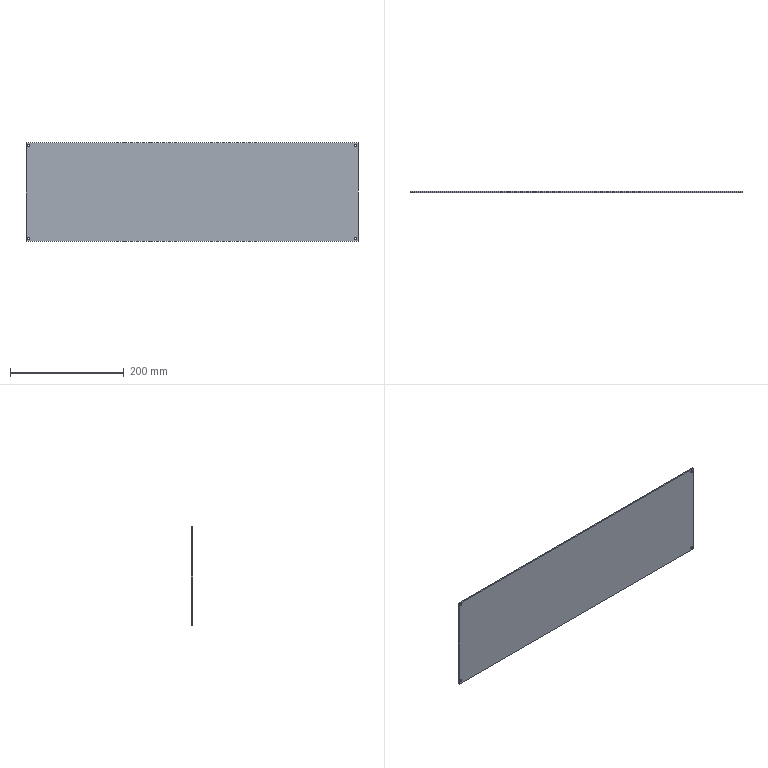Component | SolidWorks | TransformerBoxAssembly-1_ElectricalBoxTopPlate-1 | 1 solid | 14 faces | box 583 x 2 x 173 mm | volume 201617 mm3 | cylinder 8 | plane 6 | commonest cylinder face diameters 4 x8
build123d program:
from build123d import *

# Parameters (mm, degrees)
SKETCH1_W           = 583
SKETCH1_H           = 173
SKETCH1_R           = 2
BOSS_EXTRUDE1_DEPTH = 2


with BuildPart() as part:
    # Sketch1 → Boss-Extrude1 (new body)
    with BuildSketch(Plane.XY):
        with Locations((239.686, -61.336)):
            Rectangle(SKETCH1_W, SKETCH1_H)
        with Locations((-46.814, 20.164)):
            Circle(SKETCH1_R, mode=Mode.SUBTRACT)
        with Locations((-46.814, -142.836)):
            Circle(SKETCH1_R, mode=Mode.SUBTRACT)
        with Locations((526.186, 20.164)):
            Circle(SKETCH1_R, mode=Mode.SUBTRACT)
        with Locations((526.186, -142.836)):
            Circle(SKETCH1_R, mode=Mode.SUBTRACT)
    extrude(amount=BOSS_EXTRUDE1_DEPTH)


solid = part.part

# Placed as in the assembly
solid = solid.moved(Location((-831.736, 541.566, -524.683), (90, 0, 0)))
STEP:
#1=COLOUR_RGB('',0.7922,0.8196,0.9333);
#2=FILL_AREA_STYLE_COLOUR('',#1);
#3=FILL_AREA_STYLE('',(#2));
#4=SURFACE_STYLE_FILL_AREA(#3);
#5=SURFACE_SIDE_STYLE('',(#4));
#6=SURFACE_STYLE_USAGE(.BOTH.,#5);
#7=PRESENTATION_STYLE_ASSIGNMENT((#6));
#8=CARTESIAN_POINT('',(-34.51,21.243,-19.863));
#9=VERTEX_POINT('',#8);
#10=CARTESIAN_POINT('',(-34.667,21.243,-19.863));
#11=VERTEX_POINT('',#10);
#12=CARTESIAN_POINT('',(-34.589,21.243,-19.863));
#13=DIRECTION('',(-0.,-1.,-0.));
#14=DIRECTION('',(-1.,0.,0.));
#15=AXIS2_PLACEMENT_3D('',#12,#13,#14);
#16=CIRCLE('',#15,0.07874);
#17=EDGE_CURVE('',#9,#11,#16,.T.);
#18=ORIENTED_EDGE('',*,*,#17,.T.);
#19=CARTESIAN_POINT('',(-34.667,21.322,-19.863));
#20=VERTEX_POINT('',#19);
#21=CARTESIAN_POINT('',(-34.667,21.243,-19.863));
#22=DIRECTION('',(0.,1.,0.));
#23=VECTOR('',#22,39.37);
#24=LINE('',#21,#23);
#25=EDGE_CURVE('',#11,#20,#24,.T.);
#26=ORIENTED_EDGE('',*,*,#25,.T.);
#27=CARTESIAN_POINT('',(-34.51,21.322,-19.863));
#28=VERTEX_POINT('',#27);
#29=CARTESIAN_POINT('',(-34.589,21.322,-19.863));
#30=DIRECTION('',(-0.,-1.,-0.));
#31=DIRECTION('',(-1.,0.,0.));
#32=AXIS2_PLACEMENT_3D('',#29,#30,#31);
#33=CIRCLE('',#32,0.07874);
#34=EDGE_CURVE('',#28,#20,#33,.T.);
#35=ORIENTED_EDGE('',*,*,#34,.F.);
#36=CARTESIAN_POINT('',(-34.51,21.243,-19.863));
#37=DIRECTION('',(0.,1.,0.));
#38=VECTOR('',#37,39.37);
#39=LINE('',#36,#38);
#40=EDGE_CURVE('',#9,#28,#39,.T.);
#41=ORIENTED_EDGE('',*,*,#40,.F.);
#42=EDGE_LOOP('',(#18,#26,#35,#41));
#43=FACE_OUTER_BOUND('',#42,.T.);
#44=CARTESIAN_POINT('',(-34.589,21.243,-19.863));
#45=DIRECTION('',(0.,1.,0.));
#46=DIRECTION('',(1.,0.,0.));
#47=AXIS2_PLACEMENT_3D('',#44,#45,#46);
#48=CYLINDRICAL_SURFACE('',#47,0.07874);
#49=ADVANCED_FACE('',(#43),#48,.F.);
#50=CARTESIAN_POINT('',(-34.51,21.243,-26.28));
#51=VERTEX_POINT('',#50);
#52=CARTESIAN_POINT('',(-34.667,21.243,-26.28));
#53=VERTEX_POINT('',#52);
#54=CARTESIAN_POINT('',(-34.589,21.243,-26.28));
#55=DIRECTION('',(-0.,-1.,-0.));
#56=DIRECTION('',(-1.,0.,0.));
#57=AXIS2_PLACEMENT_3D('',#54,#55,#56);
#58=CIRCLE('',#57,0.07874);
#59=EDGE_CURVE('',#51,#53,#58,.T.);
#60=ORIENTED_EDGE('',*,*,#59,.T.);
#61=CARTESIAN_POINT('',(-34.667,21.322,-26.28));
#62=VERTEX_POINT('',#61);
#63=CARTESIAN_POINT('',(-34.667,21.243,-26.28));
#64=DIRECTION('',(0.,1.,0.));
#65=VECTOR('',#64,39.37);
#66=LINE('',#63,#65);
#67=EDGE_CURVE('',#53,#62,#66,.T.);
#68=ORIENTED_EDGE('',*,*,#67,.T.);
#69=CARTESIAN_POINT('',(-34.51,21.322,-26.28));
#70=VERTEX_POINT('',#69);
#71=CARTESIAN_POINT('',(-34.589,21.322,-26.28));
#72=DIRECTION('',(-0.,-1.,-0.));
#73=DIRECTION('',(-1.,0.,0.));
#74=AXIS2_PLACEMENT_3D('',#71,#72,#73);
#75=CIRCLE('',#74,0.07874);
#76=EDGE_CURVE('',#70,#62,#75,.T.);
#77=ORIENTED_EDGE('',*,*,#76,.F.);
#78=CARTESIAN_POINT('',(-34.51,21.243,-26.28));
#79=DIRECTION('',(0.,1.,0.));
#80=VECTOR('',#79,39.37);
#81=LINE('',#78,#80);
#82=EDGE_CURVE('',#51,#70,#81,.T.);
#83=ORIENTED_EDGE('',*,*,#82,.F.);
#84=EDGE_LOOP('',(#60,#68,#77,#83));
#85=FACE_OUTER_BOUND('',#84,.T.);
#86=CARTESIAN_POINT('',(-34.589,21.243,-26.28));
#87=DIRECTION('',(0.,1.,0.));
#88=DIRECTION('',(1.,0.,0.));
#89=AXIS2_PLACEMENT_3D('',#86,#87,#88);
#90=CYLINDRICAL_SURFACE('',#89,0.07874);
#91=ADVANCED_FACE('',(#85),#90,.F.);
#92=CARTESIAN_POINT('',(-11.951,21.243,-19.863));
#93=VERTEX_POINT('',#92);
#94=CARTESIAN_POINT('',(-12.108,21.243,-19.863));
#95=VERTEX_POINT('',#94);
#96=CARTESIAN_POINT('',(-12.03,21.243,-19.863));
#97=DIRECTION('',(-0.,-1.,-0.));
#98=DIRECTION('',(-1.,0.,0.));
#99=AXIS2_PLACEMENT_3D('',#96,#97,#98);
#100=CIRCLE('',#99,0.07874);
#101=EDGE_CURVE('',#93,#95,#100,.T.);
#102=ORIENTED_EDGE('',*,*,#101,.T.);
#103=CARTESIAN_POINT('',(-12.108,21.322,-19.863));
#104=VERTEX_POINT('',#103);
#105=CARTESIAN_POINT('',(-12.108,21.243,-19.863));
#106=DIRECTION('',(0.,1.,0.));
#107=VECTOR('',#106,39.37);
#108=LINE('',#105,#107);
#109=EDGE_CURVE('',#95,#104,#108,.T.);
#110=ORIENTED_EDGE('',*,*,#109,.T.);
#111=CARTESIAN_POINT('',(-11.951,21.322,-19.863));
#112=VERTEX_POINT('',#111);
#113=CARTESIAN_POINT('',(-12.03,21.322,-19.863));
#114=DIRECTION('',(-0.,-1.,-0.));
#115=DIRECTION('',(-1.,0.,0.));
#116=AXIS2_PLACEMENT_3D('',#113,#114,#115);
#117=CIRCLE('',#116,0.07874);
#118=EDGE_CURVE('',#112,#104,#117,.T.);
#119=ORIENTED_EDGE('',*,*,#118,.F.);
#120=CARTESIAN_POINT('',(-11.951,21.243,-19.863));
#121=DIRECTION('',(0.,1.,0.));
#122=VECTOR('',#121,39.37);
#123=LINE('',#120,#122);
#124=EDGE_CURVE('',#93,#112,#123,.T.);
#125=ORIENTED_EDGE('',*,*,#124,.F.);
#126=EDGE_LOOP('',(#102,#110,#119,#125));
#127=FACE_OUTER_BOUND('',#126,.T.);
#128=CARTESIAN_POINT('',(-12.03,21.243,-19.863));
#129=DIRECTION('',(0.,1.,0.));
#130=DIRECTION('',(1.,0.,0.));
#131=AXIS2_PLACEMENT_3D('',#128,#129,#130);
#132=CYLINDRICAL_SURFACE('',#131,0.07874);
#133=ADVANCED_FACE('',(#127),#132,.F.);
#134=CARTESIAN_POINT('',(-11.951,21.243,-26.28));
#135=VERTEX_POINT('',#134);
#136=CARTESIAN_POINT('',(-12.108,21.243,-26.28));
#137=VERTEX_POINT('',#136);
#138=CARTESIAN_POINT('',(-12.03,21.243,-26.28));
#139=DIRECTION('',(-0.,-1.,-0.));
#140=DIRECTION('',(-1.,0.,0.));
#141=AXIS2_PLACEMENT_3D('',#138,#139,#140);
#142=CIRCLE('',#141,0.07874);
#143=EDGE_CURVE('',#135,#137,#142,.T.);
#144=ORIENTED_EDGE('',*,*,#143,.T.);
#145=CARTESIAN_POINT('',(-12.108,21.322,-26.28));
#146=VERTEX_POINT('',#145);
#147=CARTESIAN_POINT('',(-12.108,21.243,-26.28));
#148=DIRECTION('',(0.,1.,0.));
#149=VECTOR('',#148,39.37);
#150=LINE('',#147,#149);
#151=EDGE_CURVE('',#137,#146,#150,.T.);
#152=ORIENTED_EDGE('',*,*,#151,.T.);
#153=CARTESIAN_POINT('',(-11.951,21.322,-26.28));
#154=VERTEX_POINT('',#153);
#155=CARTESIAN_POINT('',(-12.03,21.322,-26.28));
#156=DIRECTION('',(-0.,-1.,-0.));
#157=DIRECTION('',(-1.,0.,0.));
#158=AXIS2_PLACEMENT_3D('',#155,#156,#157);
#159=CIRCLE('',#158,0.07874);
#160=EDGE_CURVE('',#154,#146,#159,.T.);
#161=ORIENTED_EDGE('',*,*,#160,.F.);
#162=CARTESIAN_POINT('',(-11.951,21.243,-26.28));
#163=DIRECTION('',(0.,1.,0.));
#164=VECTOR('',#163,39.37);
#165=LINE('',#162,#164);
#166=EDGE_CURVE('',#135,#154,#165,.T.);
#167=ORIENTED_EDGE('',*,*,#166,.F.);
#168=EDGE_LOOP('',(#144,#152,#161,#167));
#169=FACE_OUTER_BOUND('',#168,.T.);
#170=CARTESIAN_POINT('',(-12.03,21.243,-26.28));
#171=DIRECTION('',(0.,1.,0.));
#172=DIRECTION('',(1.,0.,0.));
#173=AXIS2_PLACEMENT_3D('',#170,#171,#172);
#174=CYLINDRICAL_SURFACE('',#173,0.07874);
#175=ADVANCED_FACE('',(#169),#174,.F.);
#176=ORIENTED_EDGE('',*,*,#59,.F.);
#177=CARTESIAN_POINT('',(-34.589,21.243,-26.28));
#178=DIRECTION('',(-0.,-1.,-0.));
#179=DIRECTION('',(-1.,0.,0.));
#180=AXIS2_PLACEMENT_3D('',#177,#178,#179);
#181=CIRCLE('',#180,0.07874);
#182=EDGE_CURVE('',#53,#51,#181,.T.);
#183=ORIENTED_EDGE('',*,*,#182,.F.);
#184=EDGE_LOOP('',(#176,#183));
#185=FACE_BOUND('',#184,.T.);
#186=ORIENTED_EDGE('',*,*,#143,.F.);
#187=CARTESIAN_POINT('',(-12.03,21.243,-26.28));
#188=DIRECTION('',(-0.,-1.,-0.));
#189=DIRECTION('',(-1.,0.,0.));
#190=AXIS2_PLACEMENT_3D('',#187,#188,#189);
#191=CIRCLE('',#190,0.07874);
#192=EDGE_CURVE('',#137,#135,#191,.T.);
#193=ORIENTED_EDGE('',*,*,#192,.F.);
#194=EDGE_LOOP('',(#186,#193));
#195=FACE_BOUND('',#194,.T.);
#196=CARTESIAN_POINT('',(-11.833,21.243,-26.477));
#197=VERTEX_POINT('',#196);
#198=CARTESIAN_POINT('',(-11.833,21.243,-19.666));
#199=VERTEX_POINT('',#198);
#200=CARTESIAN_POINT('',(-11.833,21.243,-26.477));
#201=DIRECTION('',(0.,0.,1.));
#202=VECTOR('',#201,39.37);
#203=LINE('',#200,#202);
#204=EDGE_CURVE('',#197,#199,#203,.T.);
#205=ORIENTED_EDGE('',*,*,#204,.T.);
#206=CARTESIAN_POINT('',(-34.785,21.243,-19.666));
#207=VERTEX_POINT('',#206);
#208=CARTESIAN_POINT('',(-11.833,21.243,-19.666));
#209=DIRECTION('',(-1.,0.,0.));
#210=VECTOR('',#209,39.37);
#211=LINE('',#208,#210);
#212=EDGE_CURVE('',#199,#207,#211,.T.);
#213=ORIENTED_EDGE('',*,*,#212,.T.);
#214=CARTESIAN_POINT('',(-34.785,21.243,-26.477));
#215=VERTEX_POINT('',#214);
#216=CARTESIAN_POINT('',(-34.785,21.243,-26.477));
#217=DIRECTION('',(-0.,-0.,-1.));
#218=VECTOR('',#217,39.37);
#219=LINE('',#216,#218);
#220=EDGE_CURVE('',#207,#215,#219,.T.);
#221=ORIENTED_EDGE('',*,*,#220,.T.);
#222=CARTESIAN_POINT('',(-11.833,21.243,-26.477));
#223=DIRECTION('',(1.,-0.,-0.));
#224=VECTOR('',#223,39.37);
#225=LINE('',#222,#224);
#226=EDGE_CURVE('',#215,#197,#225,.T.);
#227=ORIENTED_EDGE('',*,*,#226,.T.);
#228=EDGE_LOOP('',(#205,#213,#221,#227));
#229=FACE_OUTER_BOUND('',#228,.T.);
#230=ORIENTED_EDGE('',*,*,#101,.F.);
#231=CARTESIAN_POINT('',(-12.03,21.243,-19.863));
#232=DIRECTION('',(-0.,-1.,-0.));
#233=DIRECTION('',(-1.,0.,0.));
#234=AXIS2_PLACEMENT_3D('',#231,#232,#233);
#235=CIRCLE('',#234,0.07874);
#236=EDGE_CURVE('',#95,#93,#235,.T.);
#237=ORIENTED_EDGE('',*,*,#236,.F.);
#238=EDGE_LOOP('',(#230,#237));
#239=FACE_BOUND('',#238,.T.);
#240=ORIENTED_EDGE('',*,*,#17,.F.);
#241=CARTESIAN_POINT('',(-34.589,21.243,-19.863));
#242=DIRECTION('',(-0.,-1.,-0.));
#243=DIRECTION('',(-1.,0.,0.));
#244=AXIS2_PLACEMENT_3D('',#241,#242,#243);
#245=CIRCLE('',#244,0.07874);
#246=EDGE_CURVE('',#11,#9,#245,.T.);
#247=ORIENTED_EDGE('',*,*,#246,.F.);
#248=EDGE_LOOP('',(#240,#247));
#249=FACE_BOUND('',#248,.T.);
#250=CARTESIAN_POINT('',(-13.873,21.243,-25.486));
#251=DIRECTION('',(-0.,-1.,-0.));
#252=DIRECTION('',(-1.,0.,0.));
#253=AXIS2_PLACEMENT_3D('',#250,#251,#252);
#254=PLANE('',#253);
#255=ADVANCED_FACE('',(#185,#195,#229,#239,#249),#254,.T.);
#256=CARTESIAN_POINT('',(-11.833,21.322,-26.477));
#257=VERTEX_POINT('',#256);
#258=CARTESIAN_POINT('',(-11.833,21.322,-19.666));
#259=VERTEX_POINT('',#258);
#260=CARTESIAN_POINT('',(-11.833,21.322,-26.477));
#261=DIRECTION('',(0.,0.,1.));
#262=VECTOR('',#261,39.37);
#263=LINE('',#260,#262);
#264=EDGE_CURVE('',#257,#259,#263,.T.);
#265=ORIENTED_EDGE('',*,*,#264,.F.);
#266=CARTESIAN_POINT('',(-34.785,21.322,-26.477));
#267=VERTEX_POINT('',#266);
#268=CARTESIAN_POINT('',(-11.833,21.322,-26.477));
#269=DIRECTION('',(1.,-0.,-0.));
#270=VECTOR('',#269,39.37);
#271=LINE('',#268,#270);
#272=EDGE_CURVE('',#267,#257,#271,.T.);
#273=ORIENTED_EDGE('',*,*,#272,.F.);
#274=CARTESIAN_POINT('',(-34.785,21.322,-19.666));
#275=VERTEX_POINT('',#274);
#276=CARTESIAN_POINT('',(-34.785,21.322,-26.477));
#277=DIRECTION('',(-0.,-0.,-1.));
#278=VECTOR('',#277,39.37);
#279=LINE('',#276,#278);
#280=EDGE_CURVE('',#275,#267,#279,.T.);
#281=ORIENTED_EDGE('',*,*,#280,.F.);
#282=CARTESIAN_POINT('',(-11.833,21.322,-19.666));
#283=DIRECTION('',(-1.,0.,0.));
#284=VECTOR('',#283,39.37);
#285=LINE('',#282,#284);
#286=EDGE_CURVE('',#259,#275,#285,.T.);
#287=ORIENTED_EDGE('',*,*,#286,.F.);
#288=EDGE_LOOP('',(#265,#273,#281,#287));
#289=FACE_OUTER_BOUND('',#288,.T.);
#290=ORIENTED_EDGE('',*,*,#160,.T.);
#291=CARTESIAN_POINT('',(-12.03,21.322,-26.28));
#292=DIRECTION('',(-0.,-1.,-0.));
#293=DIRECTION('',(-1.,0.,0.));
#294=AXIS2_PLACEMENT_3D('',#291,#292,#293);
#295=CIRCLE('',#294,0.07874);
#296=EDGE_CURVE('',#146,#154,#295,.T.);
#297=ORIENTED_EDGE('',*,*,#296,.T.);
#298=EDGE_LOOP('',(#290,#297));
#299=FACE_BOUND('',#298,.T.);
#300=ORIENTED_EDGE('',*,*,#118,.T.);
#301=CARTESIAN_POINT('',(-12.03,21.322,-19.863));
#302=DIRECTION('',(-0.,-1.,-0.));
#303=DIRECTION('',(-1.,0.,0.));
#304=AXIS2_PLACEMENT_3D('',#301,#302,#303);
#305=CIRCLE('',#304,0.07874);
#306=EDGE_CURVE('',#104,#112,#305,.T.);
#307=ORIENTED_EDGE('',*,*,#306,.T.);
#308=EDGE_LOOP('',(#300,#307));
#309=FACE_BOUND('',#308,.T.);
#310=ORIENTED_EDGE('',*,*,#76,.T.);
#311=CARTESIAN_POINT('',(-34.589,21.322,-26.28));
#312=DIRECTION('',(-0.,-1.,-0.));
#313=DIRECTION('',(-1.,0.,0.));
#314=AXIS2_PLACEMENT_3D('',#311,#312,#313);
#315=CIRCLE('',#314,0.07874);
#316=EDGE_CURVE('',#62,#70,#315,.T.);
#317=ORIENTED_EDGE('',*,*,#316,.T.);
#318=EDGE_LOOP('',(#310,#317));
#319=FACE_BOUND('',#318,.T.);
#320=ORIENTED_EDGE('',*,*,#34,.T.);
#321=CARTESIAN_POINT('',(-34.589,21.322,-19.863));
#322=DIRECTION('',(-0.,-1.,-0.));
#323=DIRECTION('',(-1.,0.,0.));
#324=AXIS2_PLACEMENT_3D('',#321,#322,#323);
#325=CIRCLE('',#324,0.07874);
#326=EDGE_CURVE('',#20,#28,#325,.T.);
#327=ORIENTED_EDGE('',*,*,#326,.T.);
#328=EDGE_LOOP('',(#320,#327));
#329=FACE_BOUND('',#328,.T.);
#330=CARTESIAN_POINT('',(-13.873,21.322,-25.486));
#331=DIRECTION('',(-0.,-1.,-0.));
#332=DIRECTION('',(-1.,0.,0.));
#333=AXIS2_PLACEMENT_3D('',#330,#331,#332);
#334=PLANE('',#333);
#335=ADVANCED_FACE('',(#289,#299,#309,#319,#329),#334,.F.);
#336=ORIENTED_EDGE('',*,*,#264,.T.);
#337=CARTESIAN_POINT('',(-11.833,21.243,-19.666));
#338=DIRECTION('',(0.,1.,0.));
#339=VECTOR('',#338,39.37);
#340=LINE('',#337,#339);
#341=EDGE_CURVE('',#199,#259,#340,.T.);
#342=ORIENTED_EDGE('',*,*,#341,.F.);
#343=ORIENTED_EDGE('',*,*,#204,.F.);
#344=CARTESIAN_POINT('',(-11.833,21.243,-26.477));
#345=DIRECTION('',(0.,1.,0.));
#346=VECTOR('',#345,39.37);
#347=LINE('',#344,#346);
#348=EDGE_CURVE('',#197,#257,#347,.T.);
#349=ORIENTED_EDGE('',*,*,#348,.T.);
#350=EDGE_LOOP('',(#336,#342,#343,#349));
#351=FACE_OUTER_BOUND('',#350,.T.);
#352=CARTESIAN_POINT('',(-11.833,21.243,-26.477));
#353=DIRECTION('',(-1.,0.,0.));
#354=DIRECTION('',(-0.,-0.,-1.));
#355=AXIS2_PLACEMENT_3D('',#352,#353,#354);
#356=PLANE('',#355);
#357=ADVANCED_FACE('',(#351),#356,.F.);
#358=ORIENTED_EDGE('',*,*,#286,.T.);
#359=CARTESIAN_POINT('',(-34.785,21.243,-19.666));
#360=DIRECTION('',(0.,1.,0.));
#361=VECTOR('',#360,39.37);
#362=LINE('',#359,#361);
#363=EDGE_CURVE('',#207,#275,#362,.T.);
#364=ORIENTED_EDGE('',*,*,#363,.F.);
#365=ORIENTED_EDGE('',*,*,#212,.F.);
#366=ORIENTED_EDGE('',*,*,#341,.T.);
#367=EDGE_LOOP('',(#358,#364,#365,#366));
#368=FACE_OUTER_BOUND('',#367,.T.);
#369=CARTESIAN_POINT('',(-11.833,21.243,-19.666));
#370=DIRECTION('',(-0.,0.,-1.));
#371=DIRECTION('',(-0.,-1.,-0.));
#372=AXIS2_PLACEMENT_3D('',#369,#370,#371);
#373=PLANE('',#372);
#374=ADVANCED_FACE('',(#368),#373,.F.);
#375=ORIENTED_EDGE('',*,*,#280,.T.);
#376=CARTESIAN_POINT('',(-34.785,21.243,-26.477));
#377=DIRECTION('',(0.,1.,0.));
#378=VECTOR('',#377,39.37);
#379=LINE('',#376,#378);
#380=EDGE_CURVE('',#215,#267,#379,.T.);
#381=ORIENTED_EDGE('',*,*,#380,.F.);
#382=ORIENTED_EDGE('',*,*,#220,.F.);
#383=ORIENTED_EDGE('',*,*,#363,.T.);
#384=EDGE_LOOP('',(#375,#381,#382,#383));
#385=FACE_OUTER_BOUND('',#384,.T.);
#386=CARTESIAN_POINT('',(-34.785,21.243,-26.477));
#387=DIRECTION('',(1.,-0.,-0.));
#388=DIRECTION('',(-0.,-1.,-0.));
#389=AXIS2_PLACEMENT_3D('',#386,#387,#388);
#390=PLANE('',#389);
#391=ADVANCED_FACE('',(#385),#390,.F.);
#392=ORIENTED_EDGE('',*,*,#272,.T.);
#393=ORIENTED_EDGE('',*,*,#348,.F.);
#394=ORIENTED_EDGE('',*,*,#226,.F.);
#395=ORIENTED_EDGE('',*,*,#380,.T.);
#396=EDGE_LOOP('',(#392,#393,#394,#395));
#397=FACE_OUTER_BOUND('',#396,.T.);
#398=CARTESIAN_POINT('',(-11.833,21.243,-26.477));
#399=DIRECTION('',(0.,-0.,1.));
#400=DIRECTION('',(0.,1.,0.));
#401=AXIS2_PLACEMENT_3D('',#398,#399,#400);
#402=PLANE('',#401);
#403=ADVANCED_FACE('',(#397),#402,.F.);
#404=ORIENTED_EDGE('',*,*,#151,.F.);
#405=ORIENTED_EDGE('',*,*,#192,.T.);
#406=ORIENTED_EDGE('',*,*,#166,.T.);
#407=ORIENTED_EDGE('',*,*,#296,.F.);
#408=EDGE_LOOP('',(#404,#405,#406,#407));
#409=FACE_OUTER_BOUND('',#408,.T.);
#410=CARTESIAN_POINT('',(-12.03,21.243,-26.28));
#411=DIRECTION('',(0.,1.,0.));
#412=DIRECTION('',(1.,0.,0.));
#413=AXIS2_PLACEMENT_3D('',#410,#411,#412);
#414=CYLINDRICAL_SURFACE('',#413,0.07874);
#415=ADVANCED_FACE('',(#409),#414,.F.);
#416=ORIENTED_EDGE('',*,*,#109,.F.);
#417=ORIENTED_EDGE('',*,*,#236,.T.);
#418=ORIENTED_EDGE('',*,*,#124,.T.);
#419=ORIENTED_EDGE('',*,*,#306,.F.);
#420=EDGE_LOOP('',(#416,#417,#418,#419));
#421=FACE_OUTER_BOUND('',#420,.T.);
#422=CARTESIAN_POINT('',(-12.03,21.243,-19.863));
#423=DIRECTION('',(0.,1.,0.));
#424=DIRECTION('',(1.,0.,0.));
#425=AXIS2_PLACEMENT_3D('',#422,#423,#424);
#426=CYLINDRICAL_SURFACE('',#425,0.07874);
#427=ADVANCED_FACE('',(#421),#426,.F.);
#428=ORIENTED_EDGE('',*,*,#67,.F.);
#429=ORIENTED_EDGE('',*,*,#182,.T.);
#430=ORIENTED_EDGE('',*,*,#82,.T.);
#431=ORIENTED_EDGE('',*,*,#316,.F.);
#432=EDGE_LOOP('',(#428,#429,#430,#431));
#433=FACE_OUTER_BOUND('',#432,.T.);
#434=CARTESIAN_POINT('',(-34.589,21.243,-26.28));
#435=DIRECTION('',(0.,1.,0.));
#436=DIRECTION('',(1.,0.,0.));
#437=AXIS2_PLACEMENT_3D('',#434,#435,#436);
#438=CYLINDRICAL_SURFACE('',#437,0.07874);
#439=ADVANCED_FACE('',(#433),#438,.F.);
#440=ORIENTED_EDGE('',*,*,#25,.F.);
#441=ORIENTED_EDGE('',*,*,#246,.T.);
#442=ORIENTED_EDGE('',*,*,#40,.T.);
#443=ORIENTED_EDGE('',*,*,#326,.F.);
#444=EDGE_LOOP('',(#440,#441,#442,#443));
#445=FACE_OUTER_BOUND('',#444,.T.);
#446=CARTESIAN_POINT('',(-34.589,21.243,-19.863));
#447=DIRECTION('',(0.,1.,0.));
#448=DIRECTION('',(1.,0.,0.));
#449=AXIS2_PLACEMENT_3D('',#446,#447,#448);
#450=CYLINDRICAL_SURFACE('',#449,0.07874);
#451=ADVANCED_FACE('',(#445),#450,.F.);
#452=CLOSED_SHELL('',(#49,#91,#133,#175,#255,#335,#357,#374,#391,#403,#415,#427,#439,#451));
#453=MANIFOLD_SOLID_BREP('',#452);
#454=STYLED_ITEM('',(#7),#453);
#455=(LENGTH_UNIT()NAMED_UNIT(*)SI_UNIT($,.METRE.));
#456=LENGTH_MEASURE_WITH_UNIT(LENGTH_MEASURE(0.0254),#455);
#457=DIMENSIONAL_EXPONENTS(1.,0.,0.,0.,0.,0.,0.);
#458=(CONVERSION_BASED_UNIT('',#456)LENGTH_UNIT()NAMED_UNIT(#457));
#459=UNCERTAINTY_MEASURE_WITH_UNIT(LENGTH_MEASURE(0.00001),#458,'','');
#460=(NAMED_UNIT(*)PLANE_ANGLE_UNIT()SI_UNIT($,.RADIAN.));
#461=(NAMED_UNIT(*)SI_UNIT($,.STERADIAN.)SOLID_ANGLE_UNIT());
#462=(GEOMETRIC_REPRESENTATION_CONTEXT(3)GLOBAL_UNCERTAINTY_ASSIGNED_CONTEXT((#459))GLOBAL_UNIT_ASSIGNED_CONTEXT((#458,#460,#461))REPRESENTATION_CONTEXT('',''));
#463=MECHANICAL_DESIGN_GEOMETRIC_PRESENTATION_REPRESENTATION('',(#454),#462);
#464=CARTESIAN_POINT('',(0.,0.,0.));
#465=DIRECTION('',(0.,0.,1.));
#466=DIRECTION('',(1.,0.,0.));
#467=AXIS2_PLACEMENT_3D('',#464,#465,#466);
#468=(LENGTH_UNIT()NAMED_UNIT(*)SI_UNIT($,.METRE.));
#469=LENGTH_MEASURE_WITH_UNIT(LENGTH_MEASURE(0.0254),#468);
#470=DIMENSIONAL_EXPONENTS(1.,0.,0.,0.,0.,0.,0.);
#471=(CONVERSION_BASED_UNIT('',#469)LENGTH_UNIT()NAMED_UNIT(#470));
#472=UNCERTAINTY_MEASURE_WITH_UNIT(LENGTH_MEASURE(0.00001),#471,'','');
#473=(NAMED_UNIT(*)PLANE_ANGLE_UNIT()SI_UNIT($,.RADIAN.));
#474=(NAMED_UNIT(*)SI_UNIT($,.STERADIAN.)SOLID_ANGLE_UNIT());
#475=(GEOMETRIC_REPRESENTATION_CONTEXT(3)GLOBAL_UNCERTAINTY_ASSIGNED_CONTEXT((#472))GLOBAL_UNIT_ASSIGNED_CONTEXT((#471,#473,#474))REPRESENTATION_CONTEXT('',''));
#476=ADVANCED_BREP_SHAPE_REPRESENTATION('',(#453,#467),#475);
#477=PRESENTATION_LAYER_ASSIGNMENT('','',(#454));